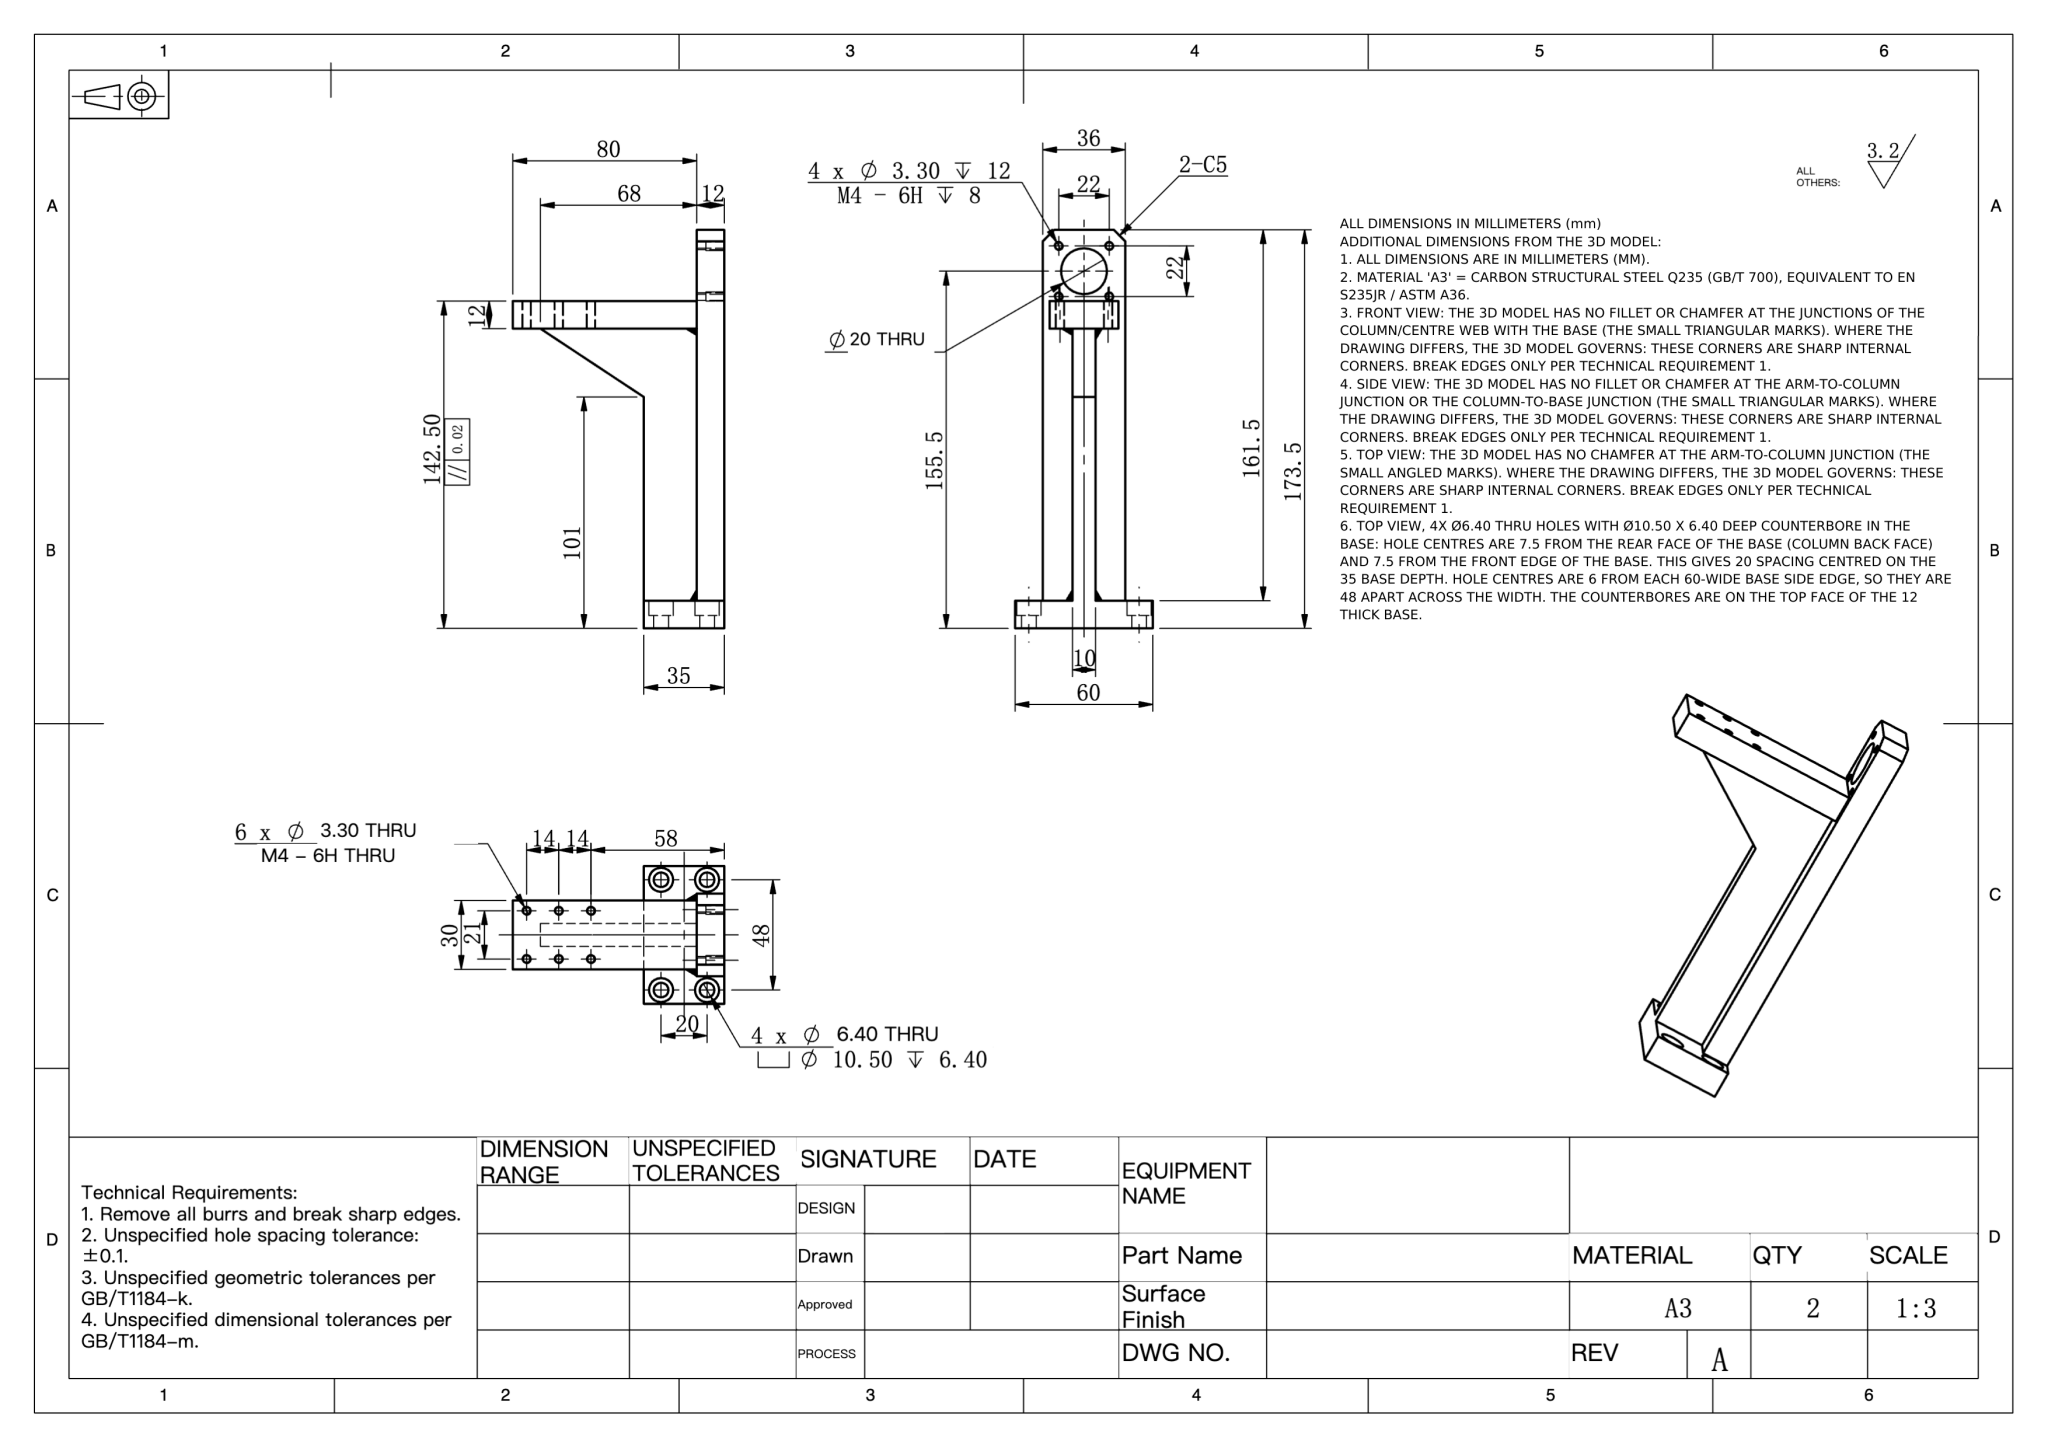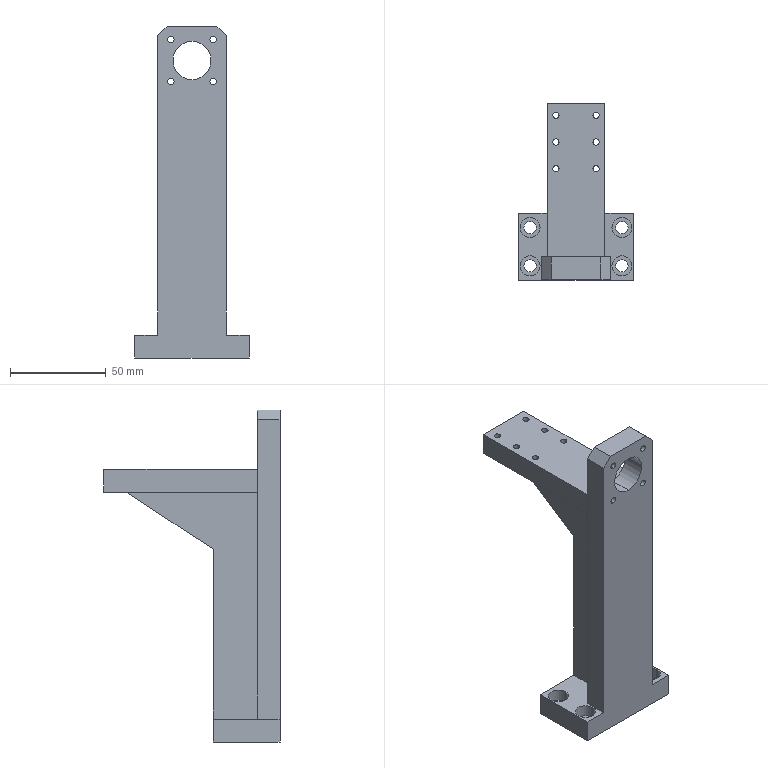Part | NX | mm | L-Shaped Support Bracket | 1 solid | 65 faces | box 60 x 92 x 173.5 mm | volume 149690 mm3 | cylinder 38 | plane 27 | commonest cylinder face diameters 3.3 x20 10.5 x8 6.4 x8 20 x2